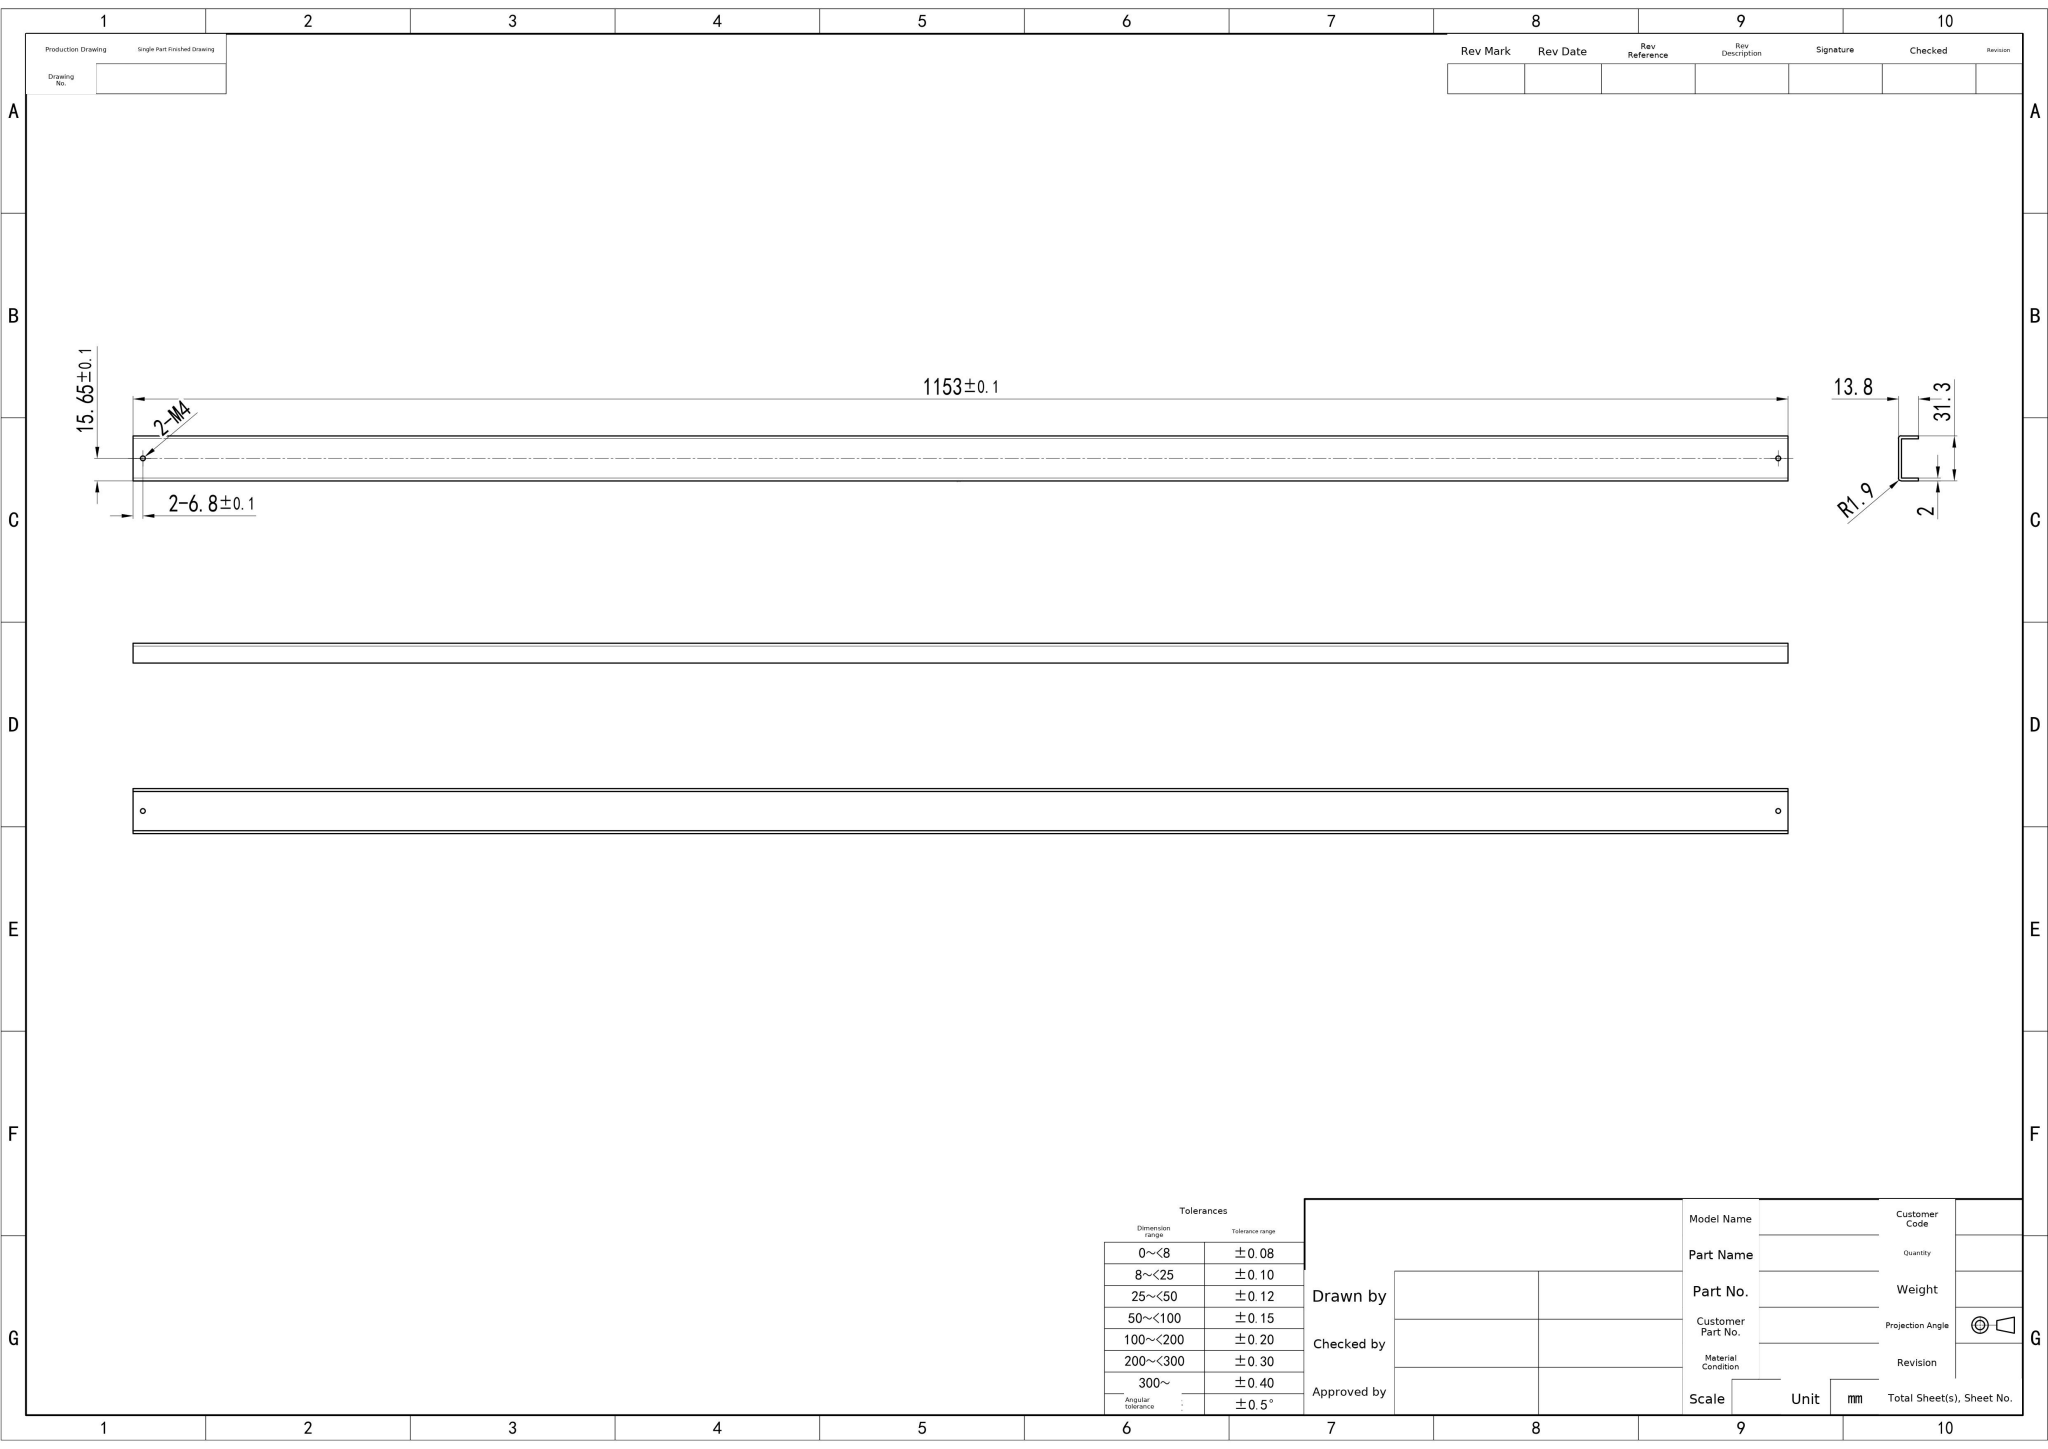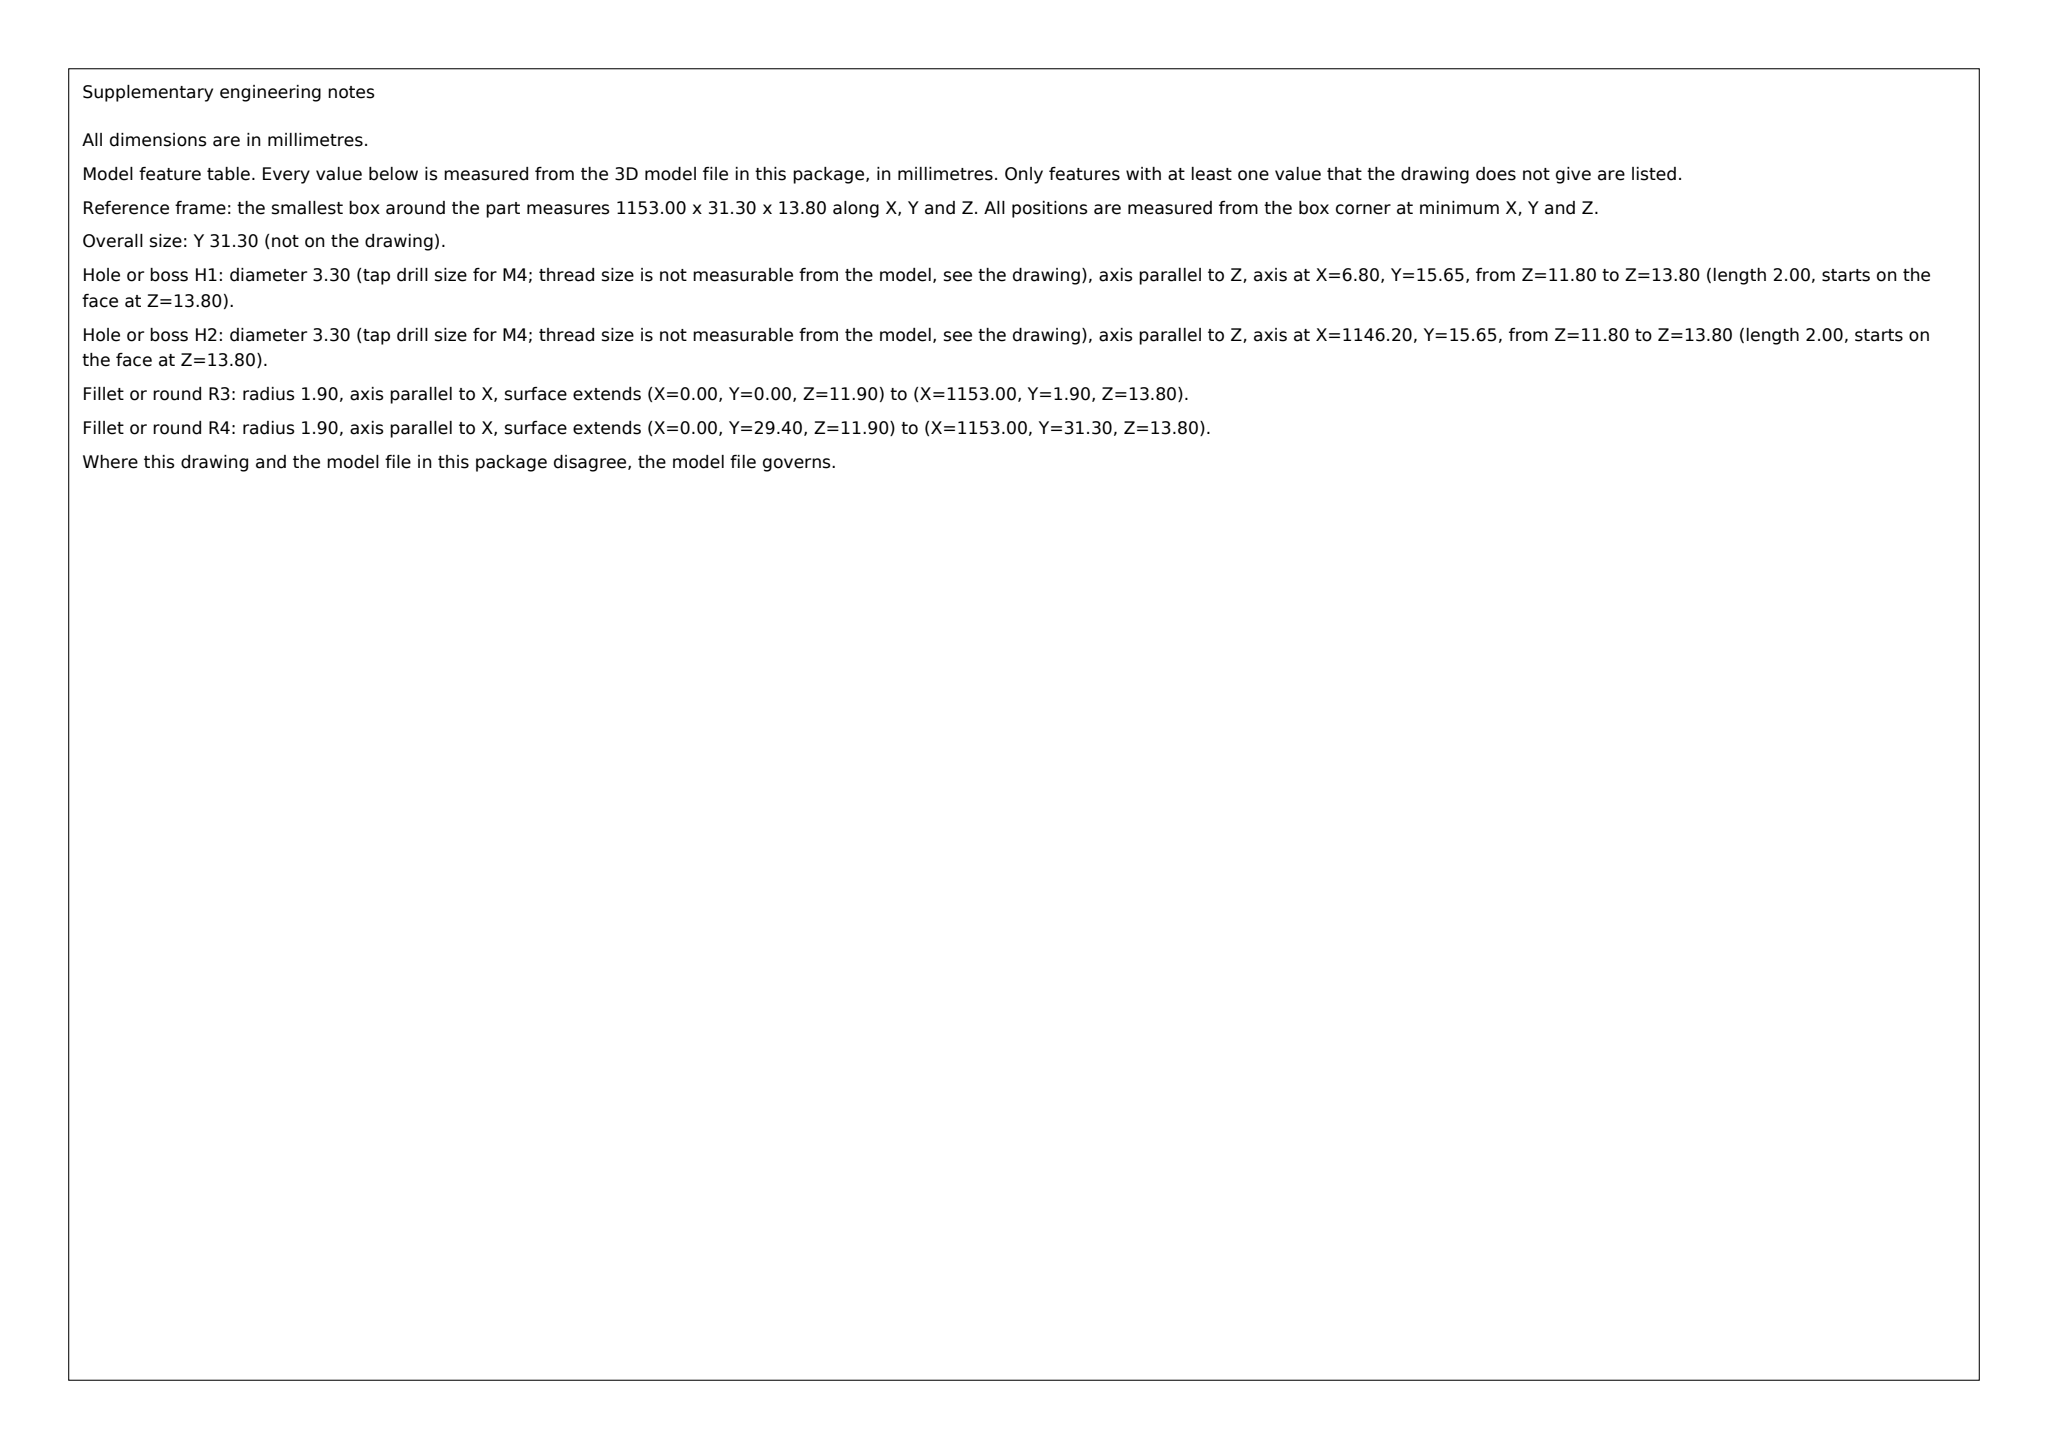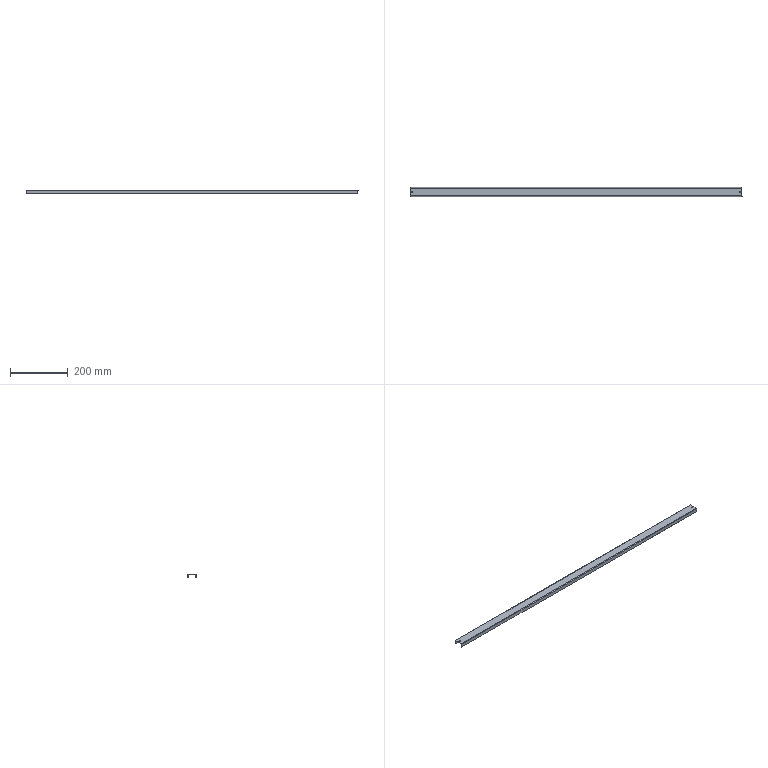Part | SolidWorks | mm | 1 solid | 16 faces | box 1153 x 31.3 x 13.8 mm | volume 124779 mm3 | plane 10 | cylinder 6 | commonest cylinder face diameters 3.3 x4 3.8 x2